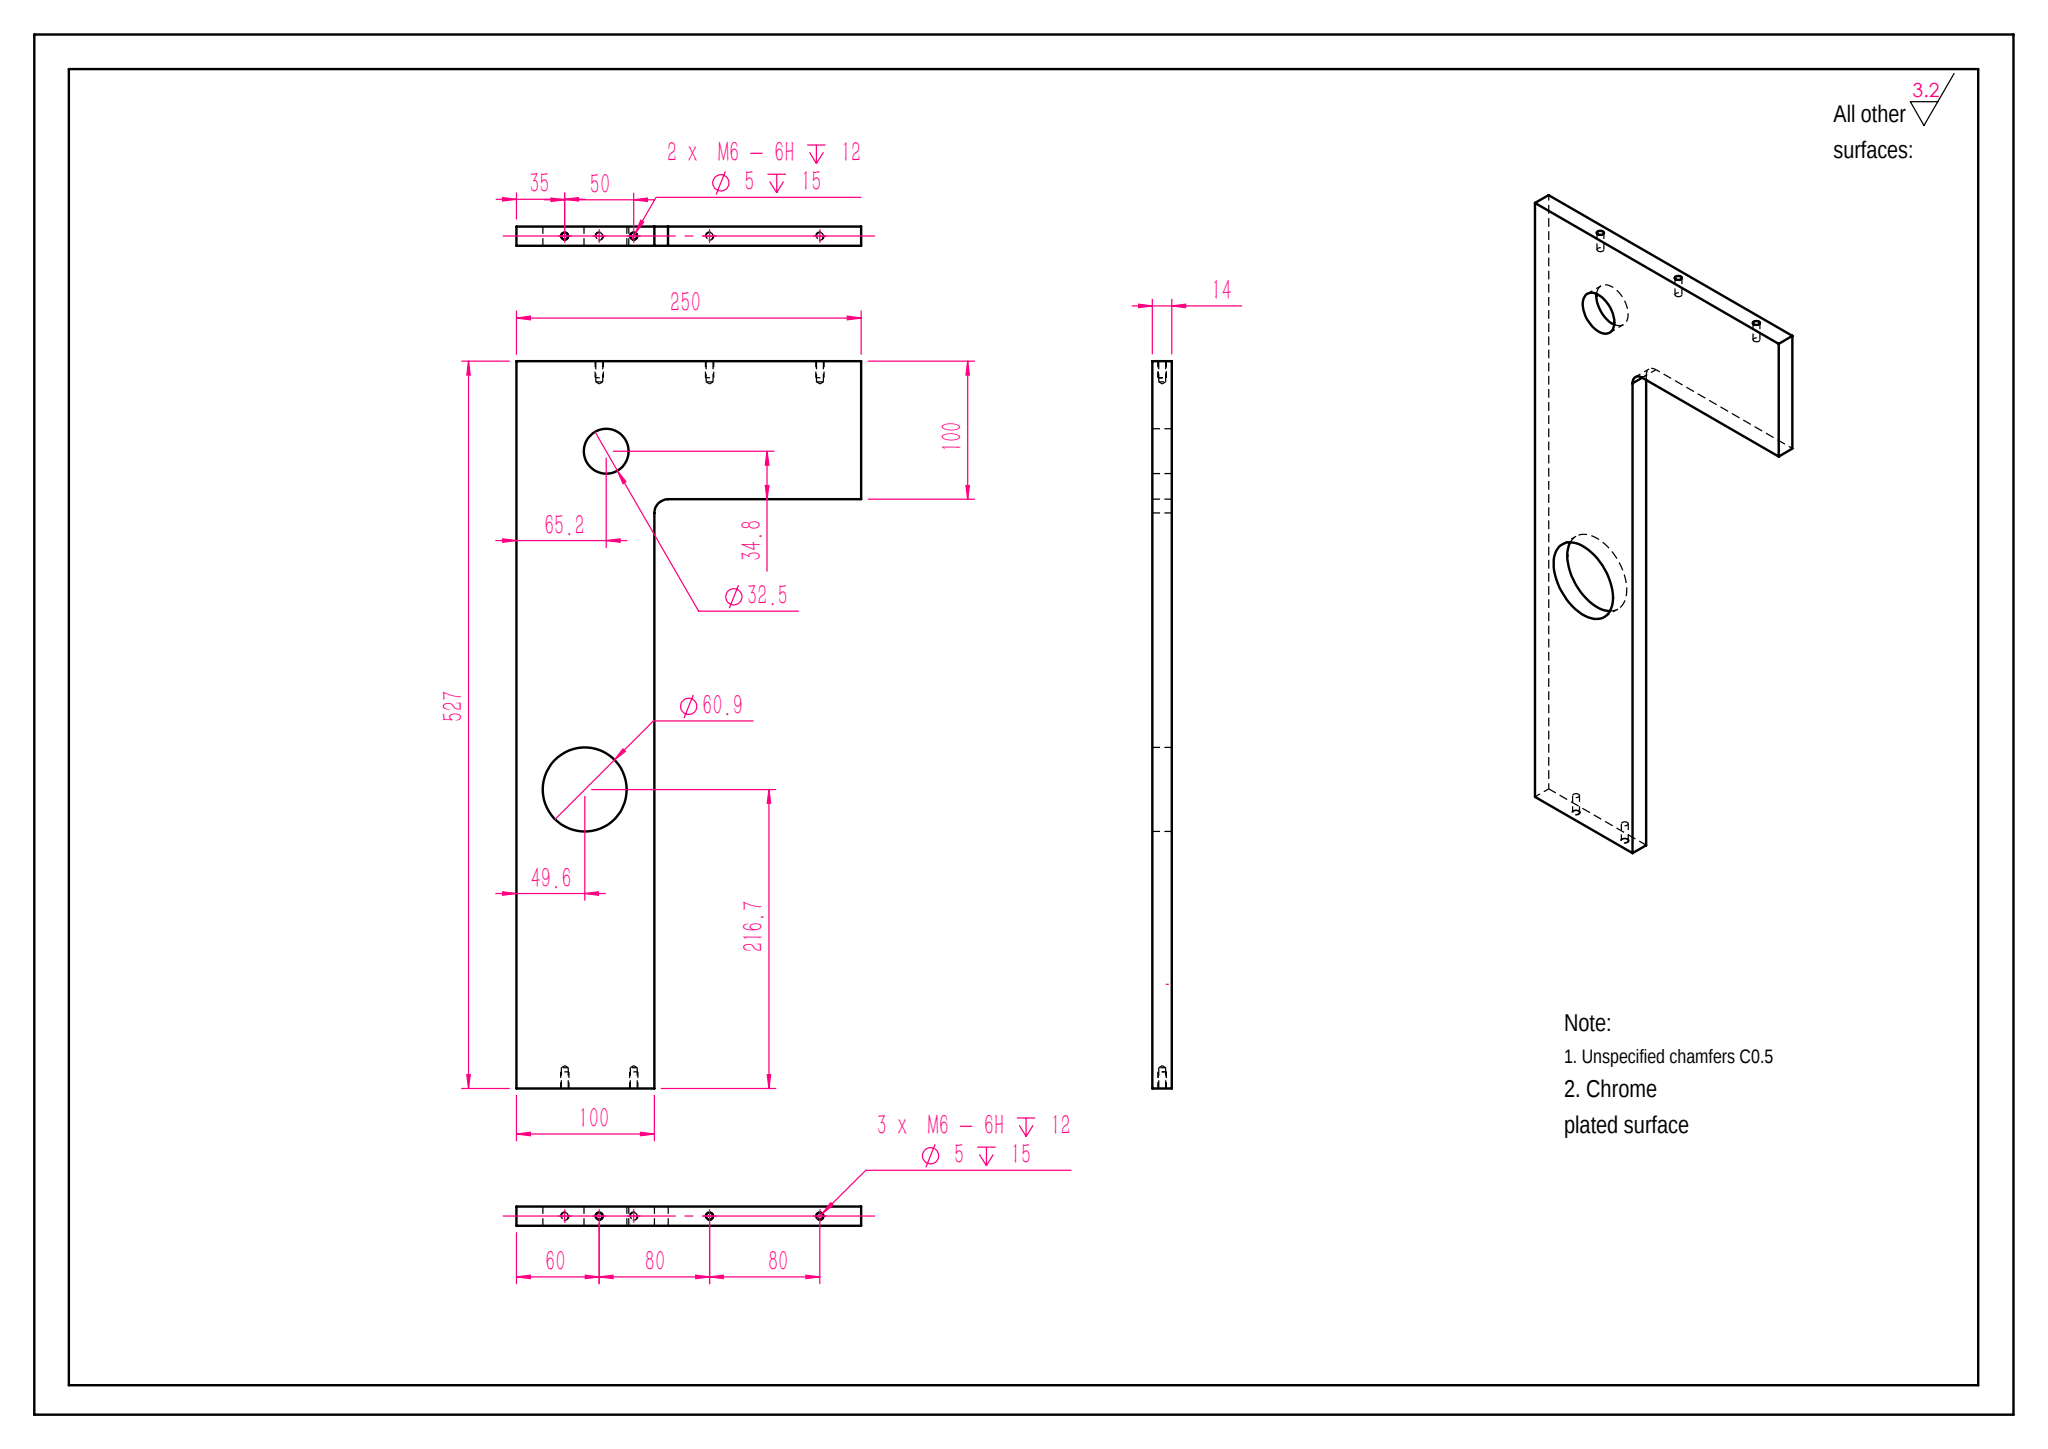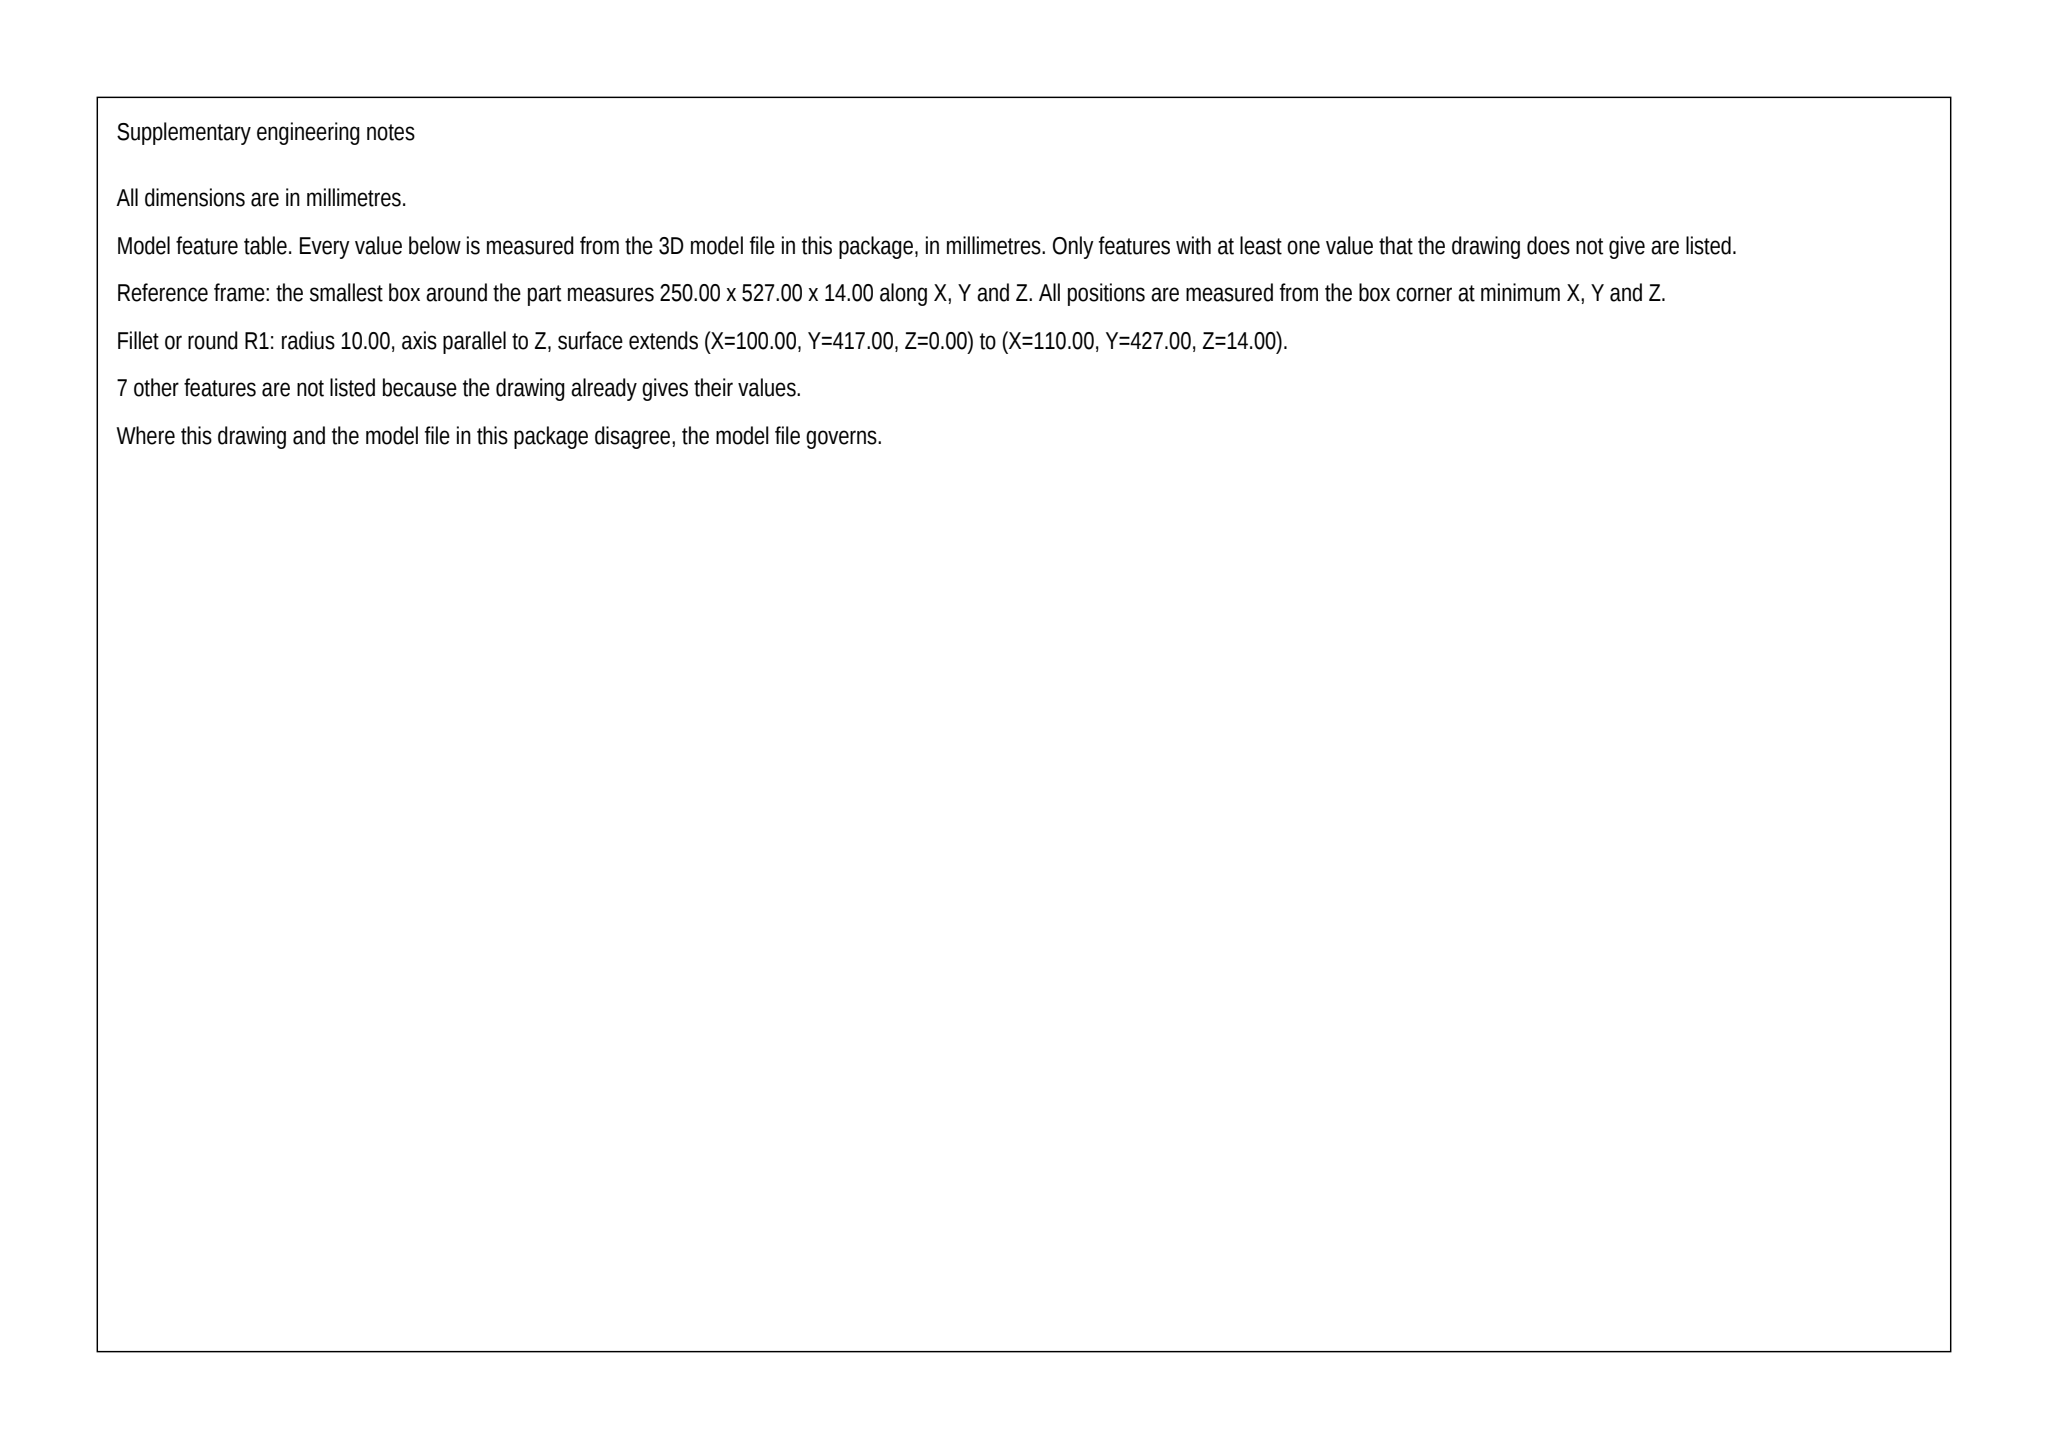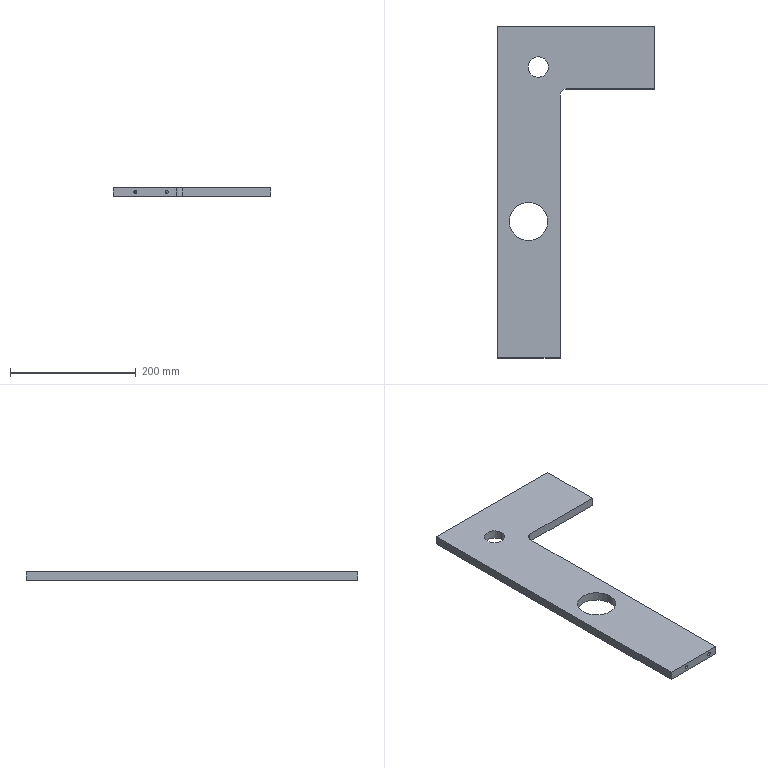Part | SolidWorks | mm | 1 solid | 33 faces | box 250 x 527 x 14 mm | volume 894206 mm3 | cylinder 15 | cone 10 | plane 8 | commonest cylinder face diameters 5 x10 60.89 x2 32.488 x2 20 x1
build123d program:
from build123d import *

# Parameters (mm, degrees)
BOSS_EXTRUDE1_DEPTH   = 7
M6_TAPPED_HOLE1_D     = 5
M6_TAPPED_HOLE1_DEPTH = 15
M6_TAPPED_HOLE1_TIP   = 1.502
M6_TAPPED_HOLE2_D     = 5
M6_TAPPED_HOLE2_DEPTH = 15
M6_TAPPED_HOLE2_TIP   = 1.502
SKETCH8_R             = 30.445
SKETCH8_R_2           = 16.244
CUT_EXTRUDE1_DEPTH    = 80


with BuildPart() as part:
    # Sketch1 → Boss-Extrude1 (new, symmetric)
    with BuildSketch(Plane.XY):
        with BuildLine():
            Line((0, 0), (100, 0))
            Line((100, 0), (100, 417))
            ThreePointArc((100, 417), (102.929, 424.071), (110, 427))
            Line((110, 427), (250, 427))
            Line((250, 427), (250, 527))
            Line((250, 527), (0, 527))
            Line((0, 527), (0, 0))
        make_face()
    extrude(amount=BOSS_EXTRUDE1_DEPTH, both=True)

    # M6 Tapped Hole1
    with Locations(Plane(origin=(0, 527, 0), x_dir=(1, 0, 0), z_dir=(0, 1, 0))):
        with Locations((60, 0), (140, 0), (220, 0)):
            Hole(M6_TAPPED_HOLE1_D / 2, depth=M6_TAPPED_HOLE1_DEPTH)
            with Locations((0, 0, -(M6_TAPPED_HOLE1_DEPTH + M6_TAPPED_HOLE1_TIP / 2))):  # 118° drill point
                Cone(0, M6_TAPPED_HOLE1_D / 2, M6_TAPPED_HOLE1_TIP, mode=Mode.SUBTRACT)

    # M6 Tapped Hole2
    with Locations(Plane(origin=(0, 0, 0), x_dir=(-1, 0, 0), z_dir=(0, -1, 0))):
        with Locations((-35, 0), (-85, 0)):
            Hole(M6_TAPPED_HOLE2_D / 2, depth=M6_TAPPED_HOLE2_DEPTH)
            with Locations((0, 0, -(M6_TAPPED_HOLE2_DEPTH + M6_TAPPED_HOLE2_TIP / 2))):  # 118° drill point
                Cone(0, M6_TAPPED_HOLE2_D / 2, M6_TAPPED_HOLE2_TIP, mode=Mode.SUBTRACT)

    # Sketch8 → Cut-Extrude1 (cut)
    with BuildSketch(Plane.XY.offset(7)):
        with Locations((49.555, 216.661)):
            Circle(SKETCH8_R)
        with Locations((65.168, 461.783)):
            Circle(SKETCH8_R_2)
    extrude(amount=-CUT_EXTRUDE1_DEPTH, mode=Mode.SUBTRACT)


solid = part.part